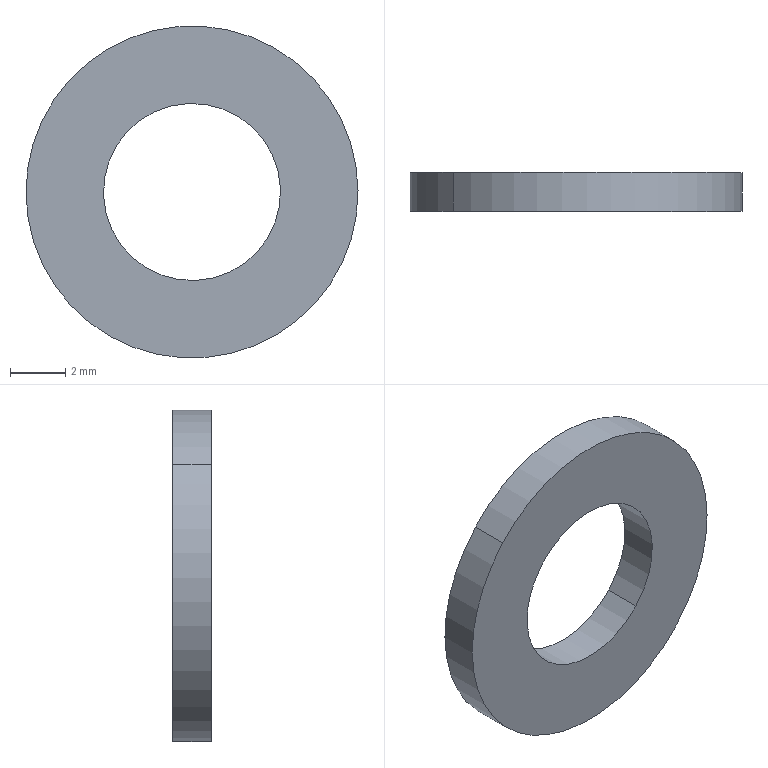Component | SolidWorks | FlatWasher_6-6 | 1 solid | 6 faces | box 12 x 1.4 x 12 mm | volume 113 mm3 | cylinder 4 | plane 2 | commonest cylinder face diameters 6.4 x2 12 x2 | material Plain Carbon Steel
build123d program:
from build123d import *

# Parameters (mm, degrees)
SKETCH1_R           = 6
SKETCH1_R_2         = 3.2
BOSS_EXTRUDE1_DEPTH = 1.4


with BuildPart() as part:
    # Sketch1 → Boss-Extrude1 (new body)
    with BuildSketch(Plane.XY):
        Circle(SKETCH1_R)
        Circle(SKETCH1_R_2, mode=Mode.SUBTRACT)
    extrude(amount=BOSS_EXTRUDE1_DEPTH)


solid = part.part

# Placed as in the assembly
solid = solid.moved(Location((-30, -23.6, 23), (90, 0, 0)))
STEP:
#1=COLOUR_RGB('',0.7922,0.8196,0.9333);
#2=FILL_AREA_STYLE_COLOUR('',#1);
#3=FILL_AREA_STYLE('',(#2));
#4=SURFACE_STYLE_FILL_AREA(#3);
#5=SURFACE_SIDE_STYLE('',(#4));
#6=SURFACE_STYLE_USAGE(.BOTH.,#5);
#7=PRESENTATION_STYLE_ASSIGNMENT((#6));
#8=CARTESIAN_POINT('',(-1.274,-0.9843,0.9903));
#9=VERTEX_POINT('',#8);
#10=CARTESIAN_POINT('',(-1.088,-0.9843,0.8207));
#11=VERTEX_POINT('',#10);
#12=CARTESIAN_POINT('',(-1.181,-0.9843,0.9055));
#13=DIRECTION('',(0.,-1.,0.));
#14=DIRECTION('',(0.7397,0.,-0.6729));
#15=AXIS2_PLACEMENT_3D('',#12,#13,#14);
#16=CIRCLE('',#15,0.126);
#17=EDGE_CURVE('',#9,#11,#16,.T.);
#18=ORIENTED_EDGE('',*,*,#17,.T.);
#19=CARTESIAN_POINT('',(-1.088,-0.9291,0.8207));
#20=VERTEX_POINT('',#19);
#21=CARTESIAN_POINT('',(-1.088,-0.9843,0.8207));
#22=DIRECTION('',(0.,1.,0.));
#23=VECTOR('',#22,39.37);
#24=LINE('',#21,#23);
#25=EDGE_CURVE('',#11,#20,#24,.T.);
#26=ORIENTED_EDGE('',*,*,#25,.T.);
#27=CARTESIAN_POINT('',(-1.274,-0.9291,0.9903));
#28=VERTEX_POINT('',#27);
#29=CARTESIAN_POINT('',(-1.181,-0.9291,0.9055));
#30=DIRECTION('',(0.,-1.,0.));
#31=DIRECTION('',(0.7397,0.,-0.6729));
#32=AXIS2_PLACEMENT_3D('',#29,#30,#31);
#33=CIRCLE('',#32,0.126);
#34=EDGE_CURVE('',#28,#20,#33,.T.);
#35=ORIENTED_EDGE('',*,*,#34,.F.);
#36=CARTESIAN_POINT('',(-1.274,-0.9843,0.9903));
#37=DIRECTION('',(0.,1.,0.));
#38=VECTOR('',#37,39.37);
#39=LINE('',#36,#38);
#40=EDGE_CURVE('',#9,#28,#39,.T.);
#41=ORIENTED_EDGE('',*,*,#40,.F.);
#42=EDGE_LOOP('',(#18,#26,#35,#41));
#43=FACE_OUTER_BOUND('',#42,.T.);
#44=CARTESIAN_POINT('',(-1.181,-0.9843,0.9055));
#45=DIRECTION('',(0.,1.,0.));
#46=DIRECTION('',(-0.7397,0.,0.6729));
#47=AXIS2_PLACEMENT_3D('',#44,#45,#46);
#48=CYLINDRICAL_SURFACE('',#47,0.126);
#49=ADVANCED_FACE('',(#43),#48,.F.);
#50=CARTESIAN_POINT('',(-1.006,-0.9843,0.7466));
#51=VERTEX_POINT('',#50);
#52=CARTESIAN_POINT('',(-1.356,-0.9843,1.064));
#53=VERTEX_POINT('',#52);
#54=CARTESIAN_POINT('',(-1.181,-0.9843,0.9055));
#55=DIRECTION('',(0.,-1.,0.));
#56=DIRECTION('',(0.7397,0.,-0.6729));
#57=AXIS2_PLACEMENT_3D('',#54,#55,#56);
#58=CIRCLE('',#57,0.2362);
#59=EDGE_CURVE('',#51,#53,#58,.T.);
#60=ORIENTED_EDGE('',*,*,#59,.F.);
#61=CARTESIAN_POINT('',(-1.006,-0.9291,0.7466));
#62=VERTEX_POINT('',#61);
#63=CARTESIAN_POINT('',(-1.006,-0.9843,0.7466));
#64=DIRECTION('',(0.,1.,0.));
#65=VECTOR('',#64,39.37);
#66=LINE('',#63,#65);
#67=EDGE_CURVE('',#51,#62,#66,.T.);
#68=ORIENTED_EDGE('',*,*,#67,.T.);
#69=CARTESIAN_POINT('',(-1.356,-0.9291,1.064));
#70=VERTEX_POINT('',#69);
#71=CARTESIAN_POINT('',(-1.181,-0.9291,0.9055));
#72=DIRECTION('',(0.,-1.,0.));
#73=DIRECTION('',(0.7397,0.,-0.6729));
#74=AXIS2_PLACEMENT_3D('',#71,#72,#73);
#75=CIRCLE('',#74,0.2362);
#76=EDGE_CURVE('',#62,#70,#75,.T.);
#77=ORIENTED_EDGE('',*,*,#76,.T.);
#78=CARTESIAN_POINT('',(-1.356,-0.9843,1.064));
#79=DIRECTION('',(0.,1.,0.));
#80=VECTOR('',#79,39.37);
#81=LINE('',#78,#80);
#82=EDGE_CURVE('',#53,#70,#81,.T.);
#83=ORIENTED_EDGE('',*,*,#82,.F.);
#84=EDGE_LOOP('',(#60,#68,#77,#83));
#85=FACE_OUTER_BOUND('',#84,.T.);
#86=CARTESIAN_POINT('',(-1.181,-0.9843,0.9055));
#87=DIRECTION('',(0.,1.,0.));
#88=DIRECTION('',(-0.7397,0.,0.6729));
#89=AXIS2_PLACEMENT_3D('',#86,#87,#88);
#90=CYLINDRICAL_SURFACE('',#89,0.2362);
#91=ADVANCED_FACE('',(#85),#90,.T.);
#92=CARTESIAN_POINT('',(-1.181,-0.9843,0.9055));
#93=DIRECTION('',(0.,-1.,0.));
#94=DIRECTION('',(0.7397,0.,-0.6729));
#95=AXIS2_PLACEMENT_3D('',#92,#93,#94);
#96=CIRCLE('',#95,0.2362);
#97=EDGE_CURVE('',#53,#51,#96,.T.);
#98=ORIENTED_EDGE('',*,*,#97,.T.);
#99=ORIENTED_EDGE('',*,*,#59,.T.);
#100=EDGE_LOOP('',(#98,#99));
#101=FACE_OUTER_BOUND('',#100,.T.);
#102=ORIENTED_EDGE('',*,*,#17,.F.);
#103=CARTESIAN_POINT('',(-1.181,-0.9843,0.9055));
#104=DIRECTION('',(0.,-1.,0.));
#105=DIRECTION('',(0.7397,0.,-0.6729));
#106=AXIS2_PLACEMENT_3D('',#103,#104,#105);
#107=CIRCLE('',#106,0.126);
#108=EDGE_CURVE('',#11,#9,#107,.T.);
#109=ORIENTED_EDGE('',*,*,#108,.F.);
#110=EDGE_LOOP('',(#102,#109));
#111=FACE_BOUND('',#110,.T.);
#112=CARTESIAN_POINT('',(-1.181,-0.9843,0.9055));
#113=DIRECTION('',(0.,-1.,0.));
#114=DIRECTION('',(0.7397,0.,-0.6729));
#115=AXIS2_PLACEMENT_3D('',#112,#113,#114);
#116=PLANE('',#115);
#117=ADVANCED_FACE('',(#101,#111),#116,.T.);
#118=CARTESIAN_POINT('',(-1.181,-0.9291,0.9055));
#119=DIRECTION('',(0.,-1.,0.));
#120=DIRECTION('',(0.7397,0.,-0.6729));
#121=AXIS2_PLACEMENT_3D('',#118,#119,#120);
#122=CIRCLE('',#121,0.2362);
#123=EDGE_CURVE('',#70,#62,#122,.T.);
#124=ORIENTED_EDGE('',*,*,#123,.F.);
#125=ORIENTED_EDGE('',*,*,#76,.F.);
#126=EDGE_LOOP('',(#124,#125));
#127=FACE_OUTER_BOUND('',#126,.T.);
#128=ORIENTED_EDGE('',*,*,#34,.T.);
#129=CARTESIAN_POINT('',(-1.181,-0.9291,0.9055));
#130=DIRECTION('',(0.,-1.,0.));
#131=DIRECTION('',(0.7397,0.,-0.6729));
#132=AXIS2_PLACEMENT_3D('',#129,#130,#131);
#133=CIRCLE('',#132,0.126);
#134=EDGE_CURVE('',#20,#28,#133,.T.);
#135=ORIENTED_EDGE('',*,*,#134,.T.);
#136=EDGE_LOOP('',(#128,#135));
#137=FACE_BOUND('',#136,.T.);
#138=CARTESIAN_POINT('',(-1.181,-0.9291,0.9055));
#139=DIRECTION('',(0.,-1.,0.));
#140=DIRECTION('',(0.7397,0.,-0.6729));
#141=AXIS2_PLACEMENT_3D('',#138,#139,#140);
#142=PLANE('',#141);
#143=ADVANCED_FACE('',(#127,#137),#142,.F.);
#144=ORIENTED_EDGE('',*,*,#67,.F.);
#145=ORIENTED_EDGE('',*,*,#97,.F.);
#146=ORIENTED_EDGE('',*,*,#82,.T.);
#147=ORIENTED_EDGE('',*,*,#123,.T.);
#148=EDGE_LOOP('',(#144,#145,#146,#147));
#149=FACE_OUTER_BOUND('',#148,.T.);
#150=CARTESIAN_POINT('',(-1.181,-0.9843,0.9055));
#151=DIRECTION('',(0.,1.,0.));
#152=DIRECTION('',(-0.7397,0.,0.6729));
#153=AXIS2_PLACEMENT_3D('',#150,#151,#152);
#154=CYLINDRICAL_SURFACE('',#153,0.2362);
#155=ADVANCED_FACE('',(#149),#154,.T.);
#156=ORIENTED_EDGE('',*,*,#25,.F.);
#157=ORIENTED_EDGE('',*,*,#108,.T.);
#158=ORIENTED_EDGE('',*,*,#40,.T.);
#159=ORIENTED_EDGE('',*,*,#134,.F.);
#160=EDGE_LOOP('',(#156,#157,#158,#159));
#161=FACE_OUTER_BOUND('',#160,.T.);
#162=CARTESIAN_POINT('',(-1.181,-0.9843,0.9055));
#163=DIRECTION('',(0.,1.,0.));
#164=DIRECTION('',(-0.7397,0.,0.6729));
#165=AXIS2_PLACEMENT_3D('',#162,#163,#164);
#166=CYLINDRICAL_SURFACE('',#165,0.126);
#167=ADVANCED_FACE('',(#161),#166,.F.);
#168=CLOSED_SHELL('',(#49,#91,#117,#143,#155,#167));
#169=MANIFOLD_SOLID_BREP('',#168);
#170=STYLED_ITEM('',(#7),#169);
#171=PRESENTATION_LAYER_ASSIGNMENT('','',(#170));
#172=(LENGTH_UNIT()NAMED_UNIT(*)SI_UNIT($,.METRE.));
#173=LENGTH_MEASURE_WITH_UNIT(LENGTH_MEASURE(0.0254),#172);
#174=DIMENSIONAL_EXPONENTS(1.,0.,0.,0.,0.,0.,0.);
#175=(CONVERSION_BASED_UNIT('',#173)LENGTH_UNIT()NAMED_UNIT(#174));
#176=UNCERTAINTY_MEASURE_WITH_UNIT(LENGTH_MEASURE(0.00001),#175,'','');
#177=(NAMED_UNIT(*)PLANE_ANGLE_UNIT()SI_UNIT($,.RADIAN.));
#178=(NAMED_UNIT(*)SI_UNIT($,.STERADIAN.)SOLID_ANGLE_UNIT());
#179=(GEOMETRIC_REPRESENTATION_CONTEXT(3)GLOBAL_UNCERTAINTY_ASSIGNED_CONTEXT((#176))GLOBAL_UNIT_ASSIGNED_CONTEXT((#175,#177,#178))REPRESENTATION_CONTEXT('',''));
#180=MECHANICAL_DESIGN_GEOMETRIC_PRESENTATION_REPRESENTATION('',(#170),#179);
#181=CARTESIAN_POINT('',(0.,0.,0.));
#182=DIRECTION('',(0.,0.,1.));
#183=DIRECTION('',(1.,0.,0.));
#184=AXIS2_PLACEMENT_3D('',#181,#182,#183);
#185=(LENGTH_UNIT()NAMED_UNIT(*)SI_UNIT($,.METRE.));
#186=LENGTH_MEASURE_WITH_UNIT(LENGTH_MEASURE(0.0254),#185);
#187=DIMENSIONAL_EXPONENTS(1.,0.,0.,0.,0.,0.,0.);
#188=(CONVERSION_BASED_UNIT('',#186)LENGTH_UNIT()NAMED_UNIT(#187));
#189=UNCERTAINTY_MEASURE_WITH_UNIT(LENGTH_MEASURE(0.00001),#188,'','');
#190=(NAMED_UNIT(*)PLANE_ANGLE_UNIT()SI_UNIT($,.RADIAN.));
#191=(NAMED_UNIT(*)SI_UNIT($,.STERADIAN.)SOLID_ANGLE_UNIT());
#192=(GEOMETRIC_REPRESENTATION_CONTEXT(3)GLOBAL_UNCERTAINTY_ASSIGNED_CONTEXT((#189))GLOBAL_UNIT_ASSIGNED_CONTEXT((#188,#190,#191))REPRESENTATION_CONTEXT('',''));
#193=ADVANCED_BREP_SHAPE_REPRESENTATION('',(#169,#184),#192);